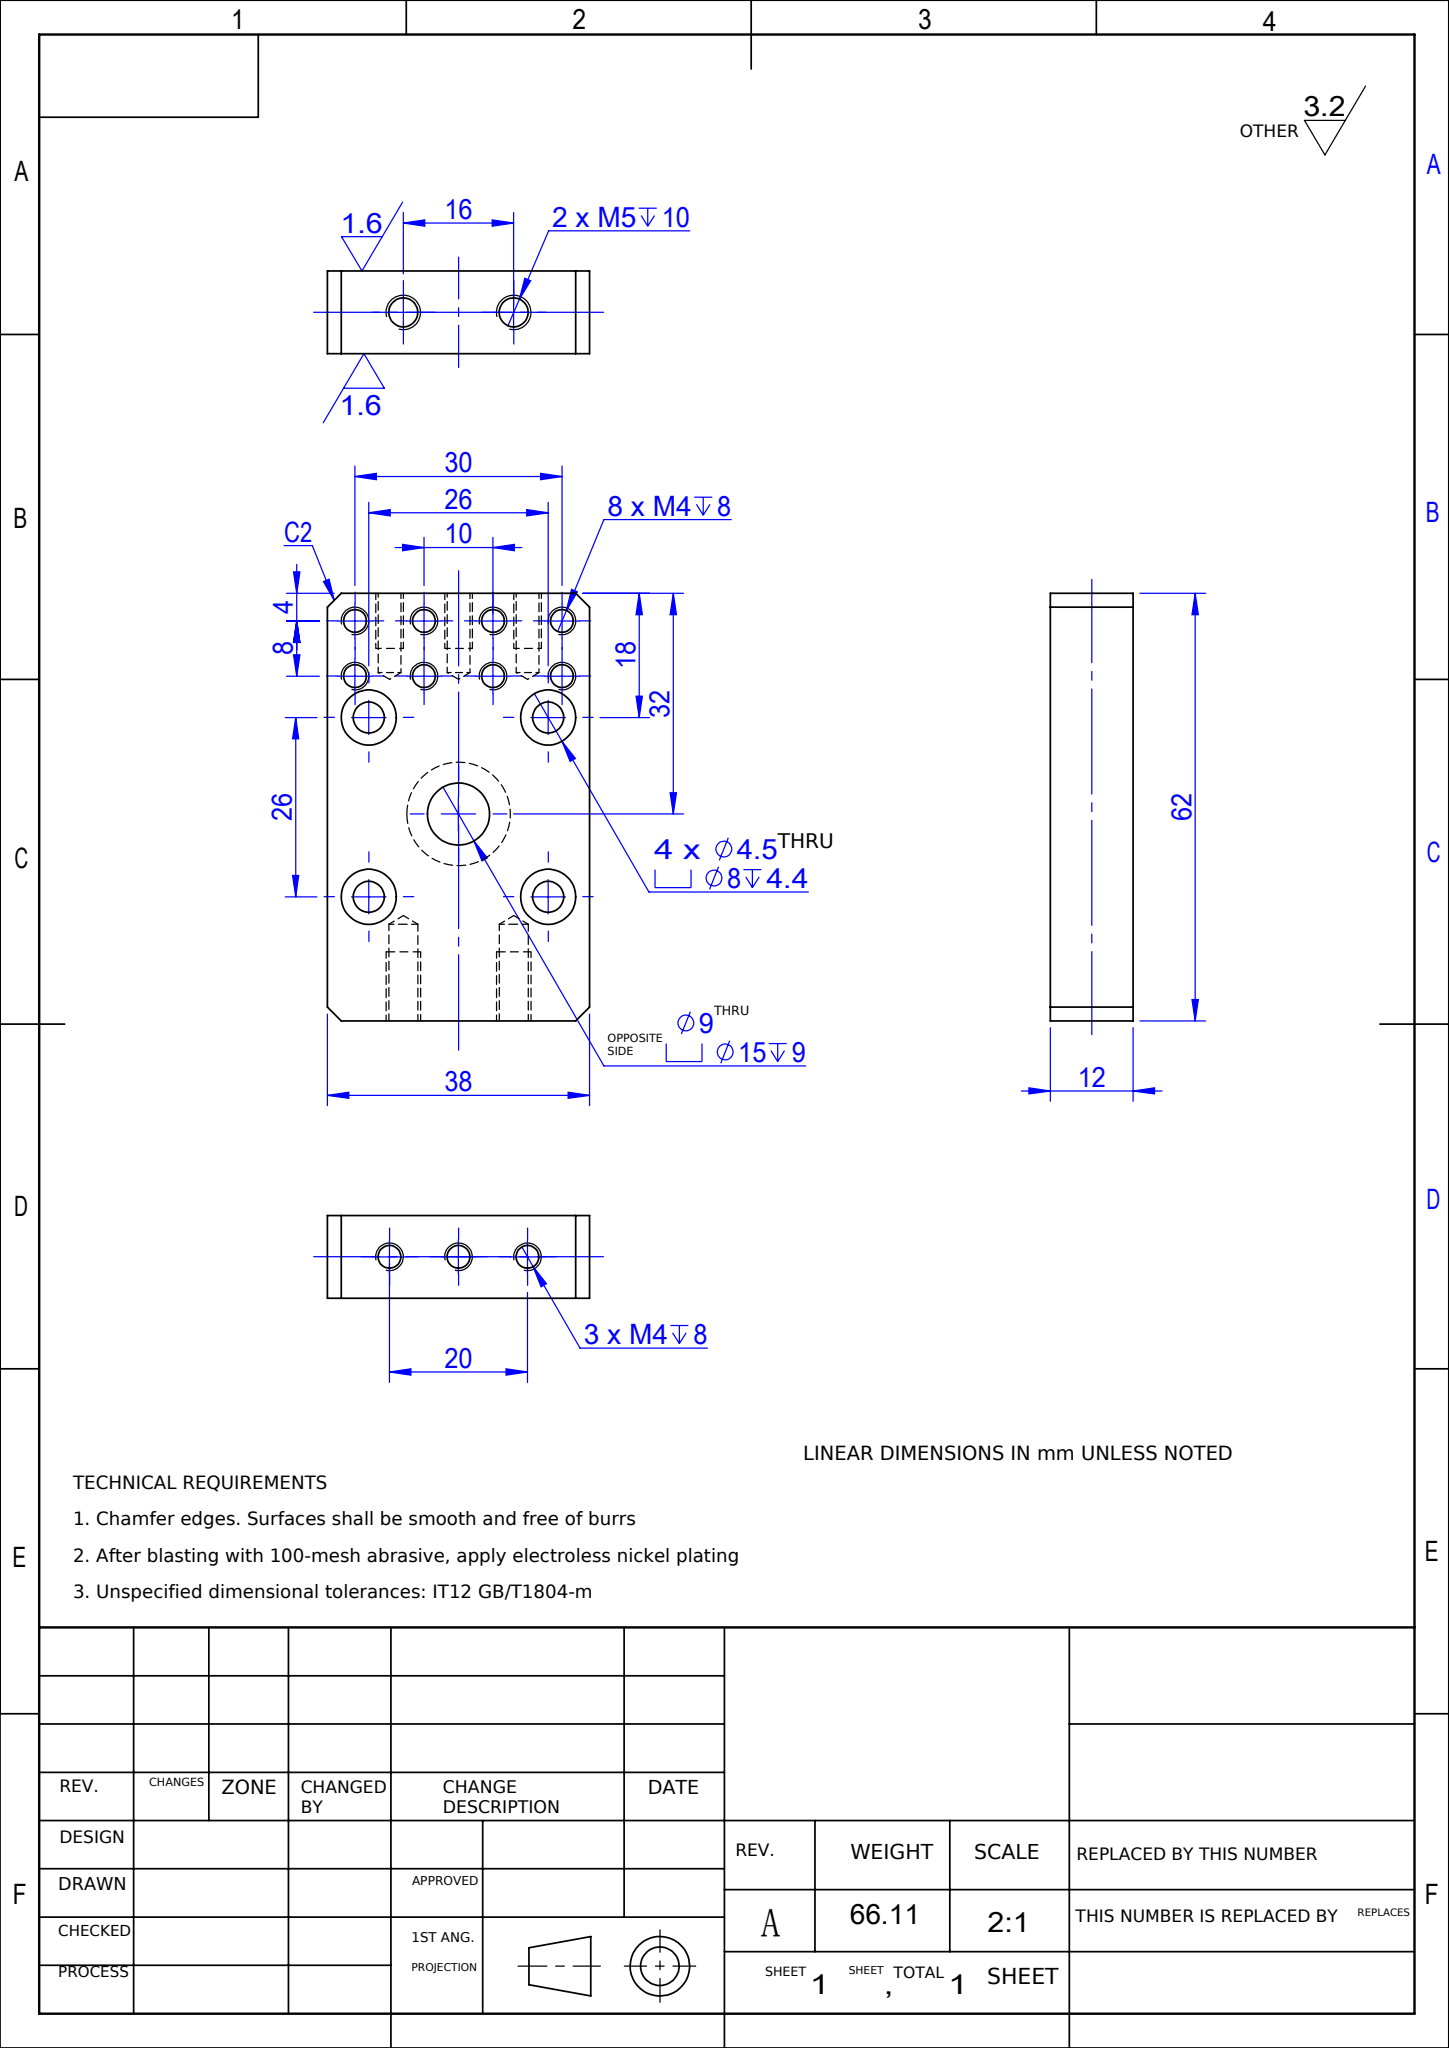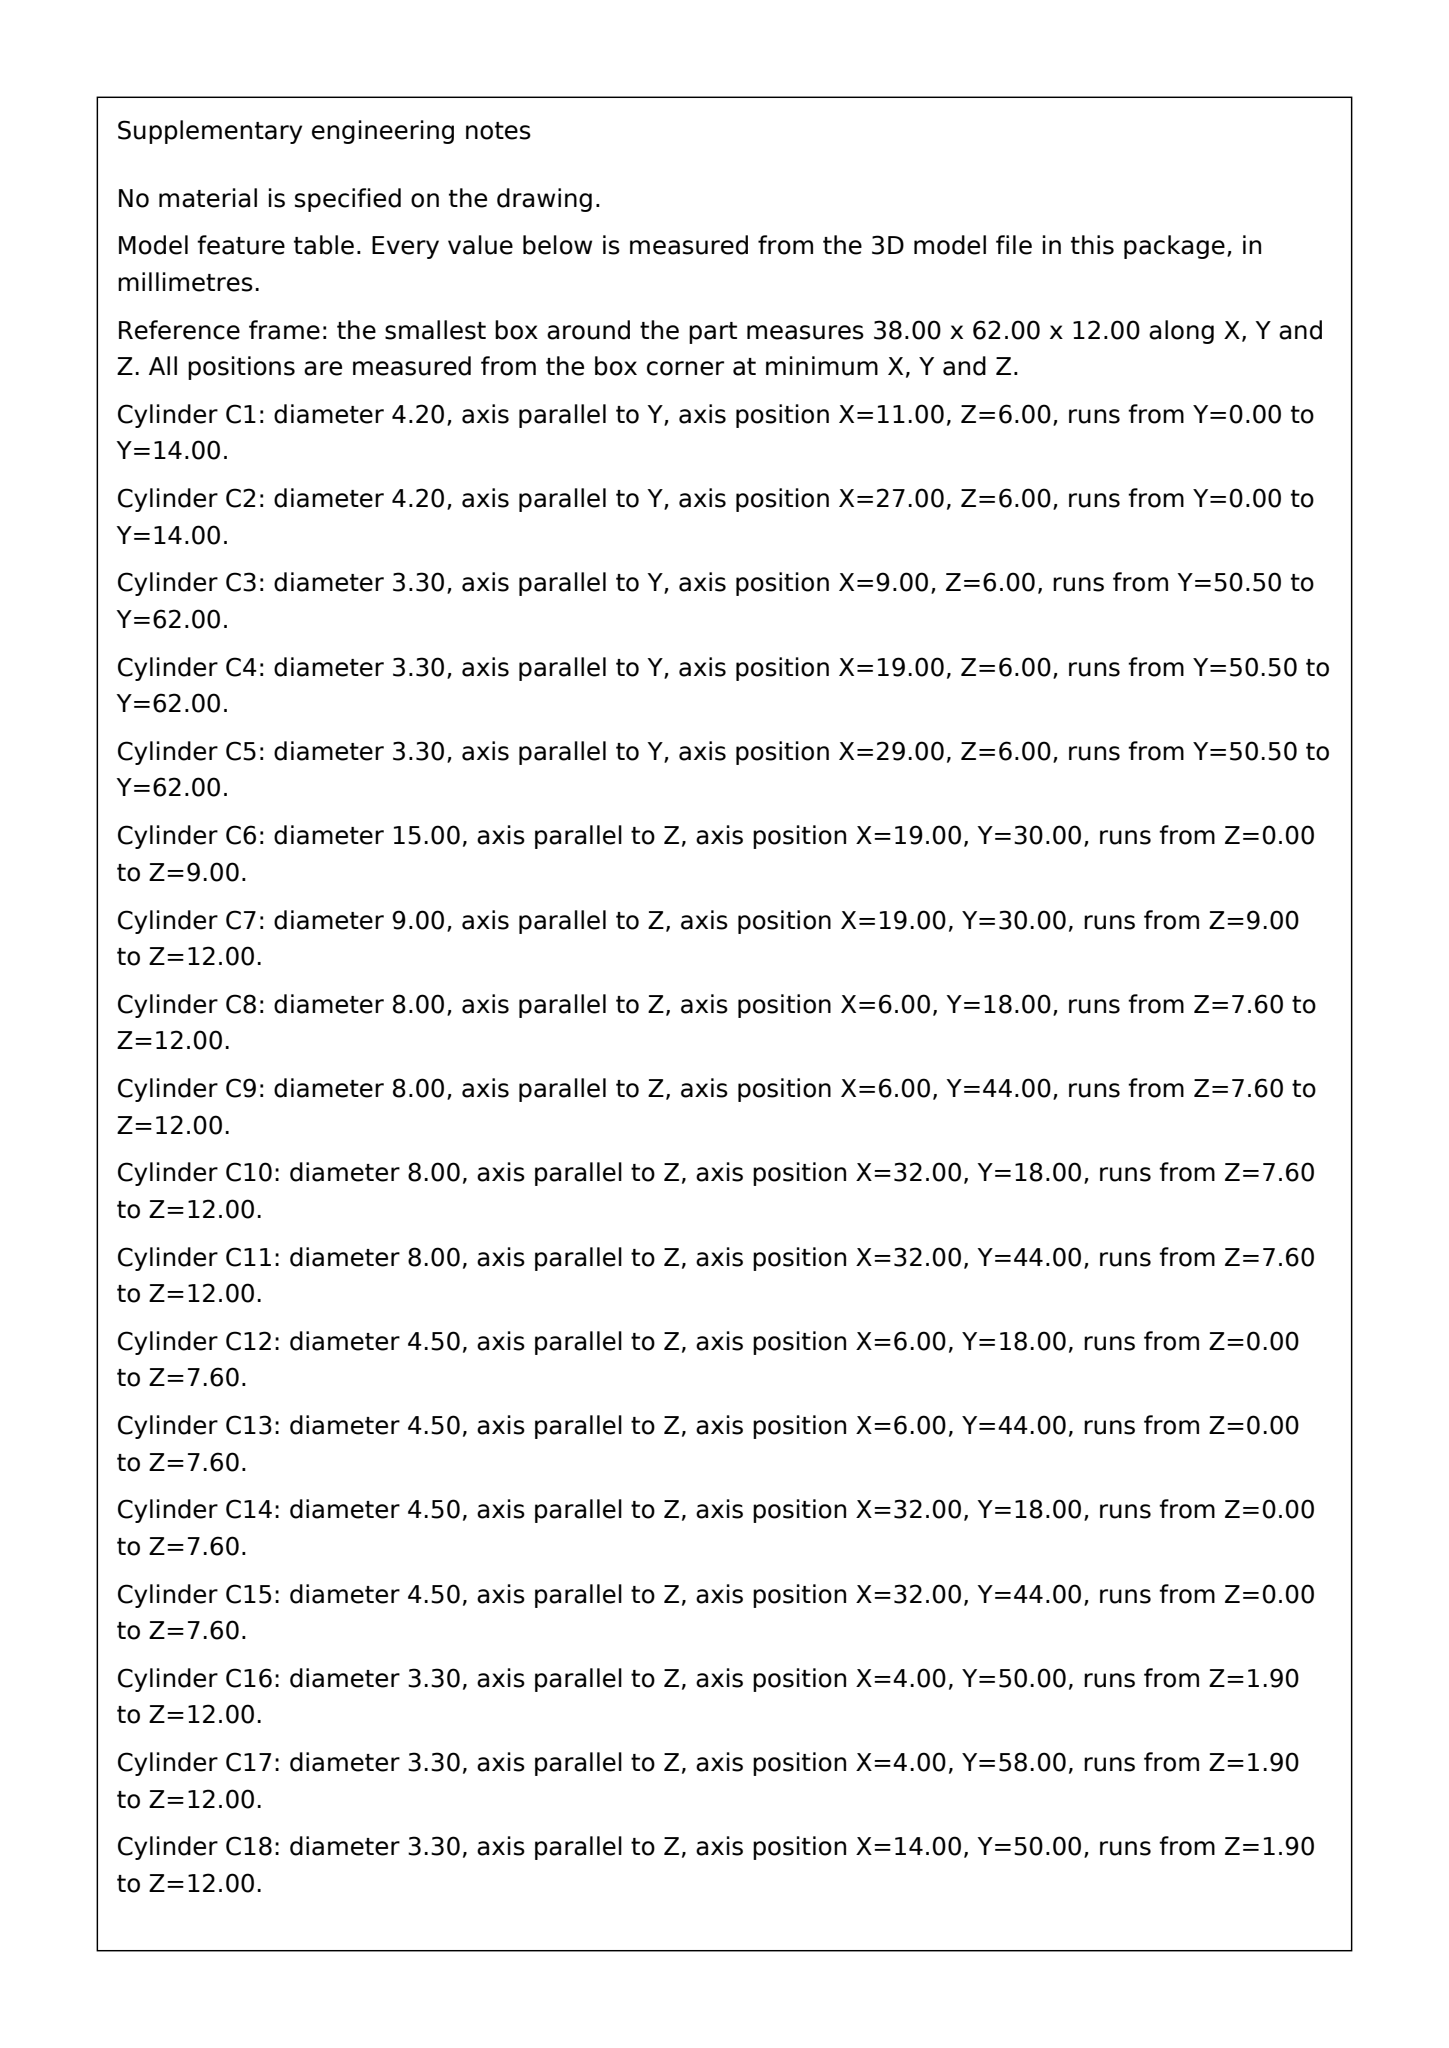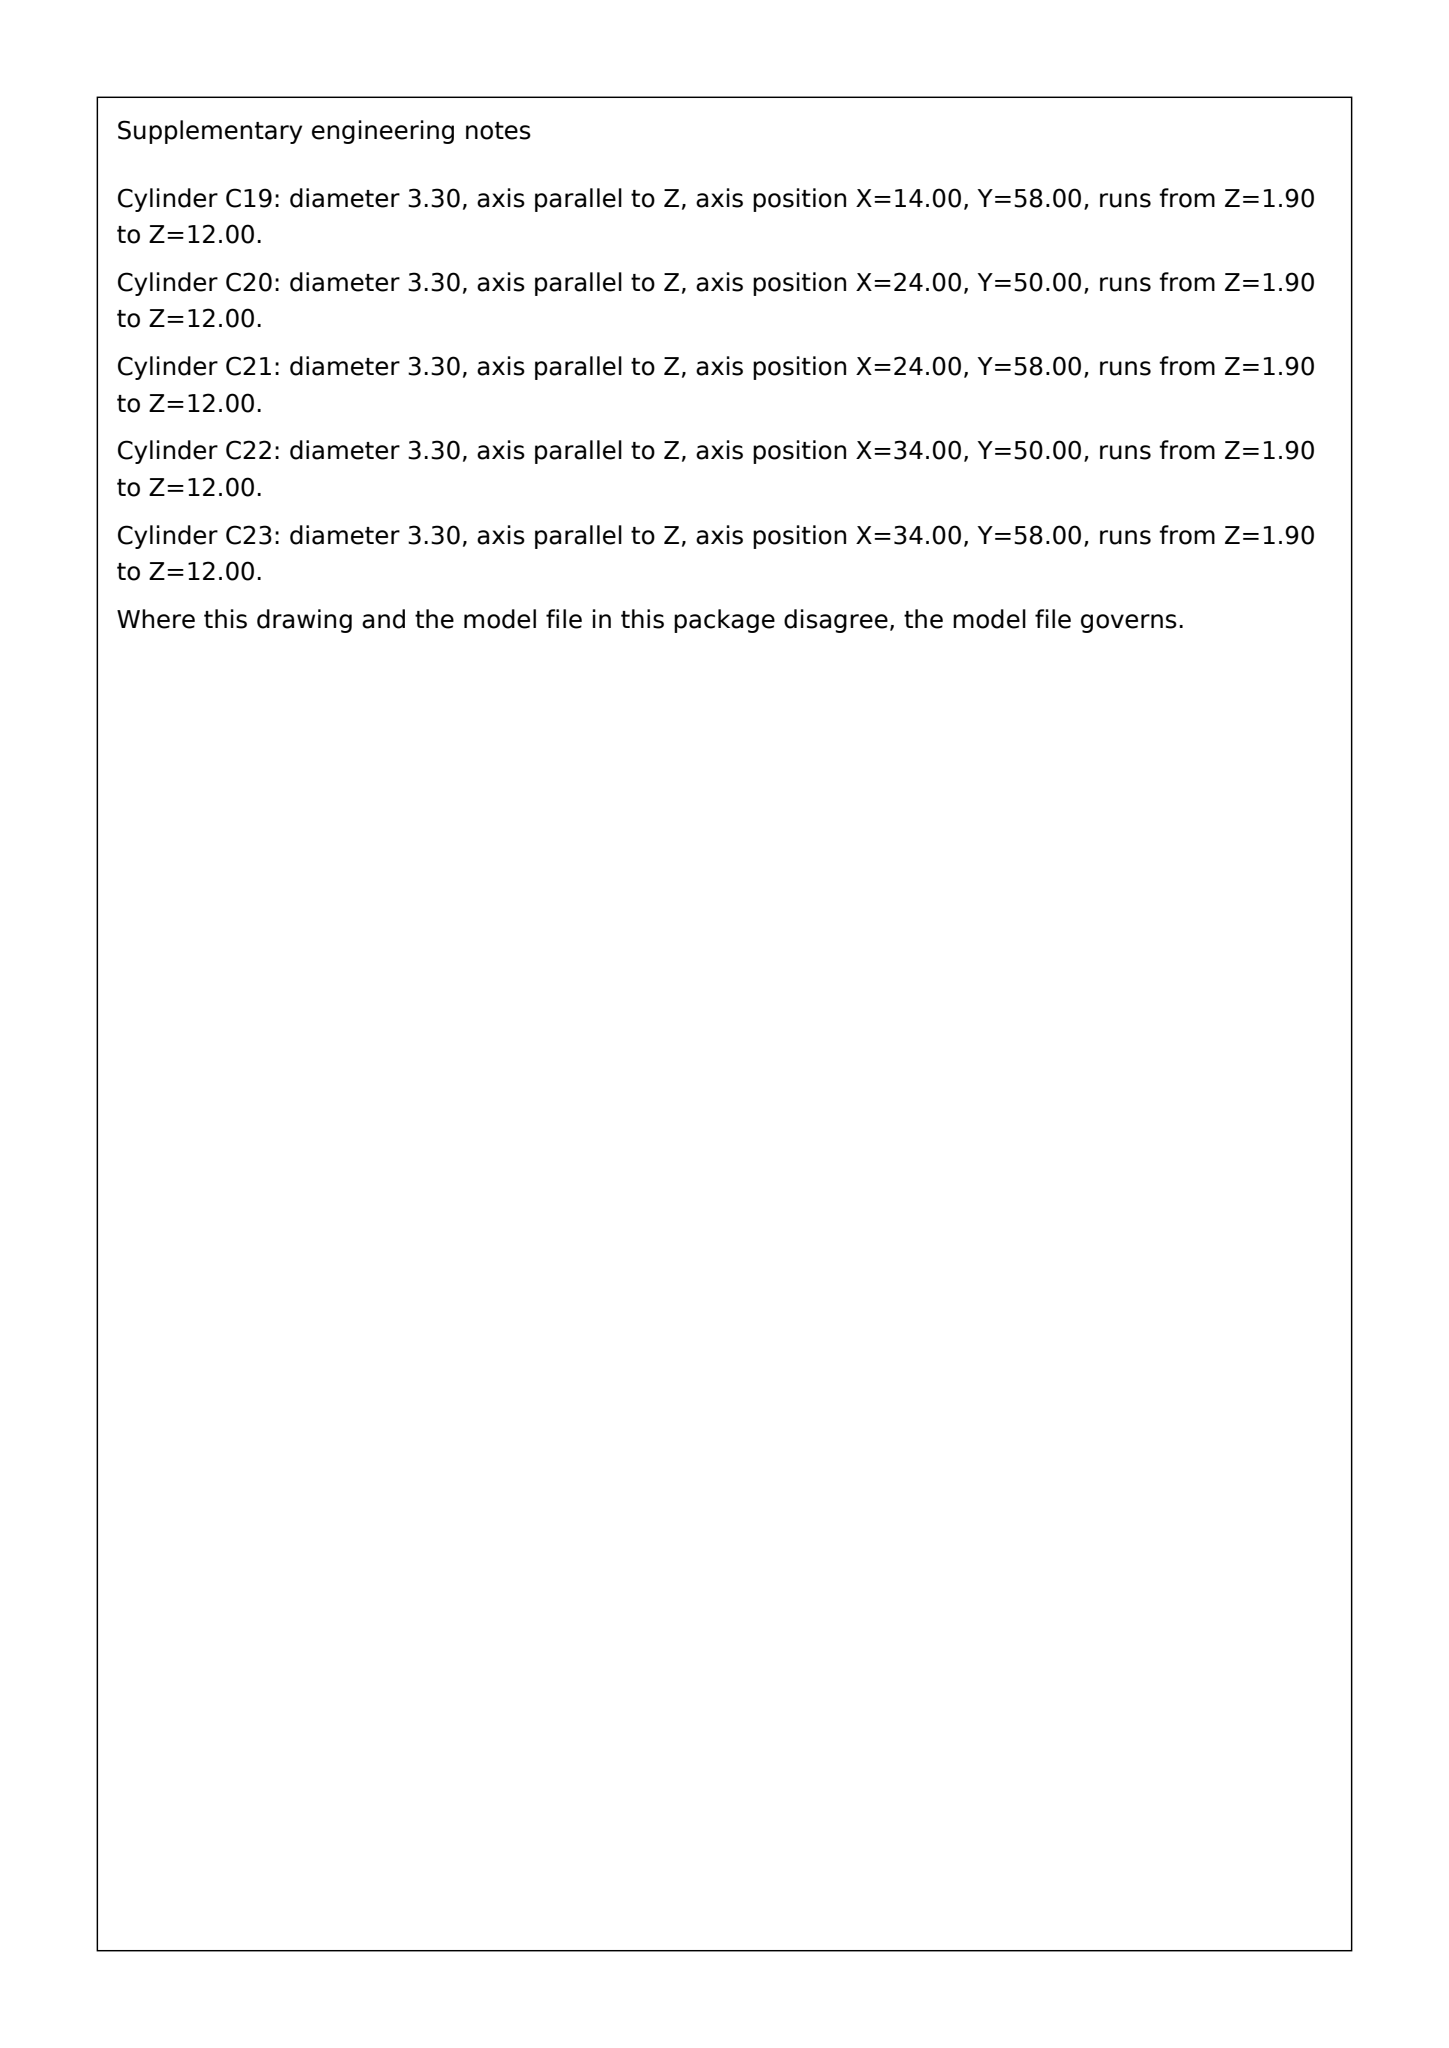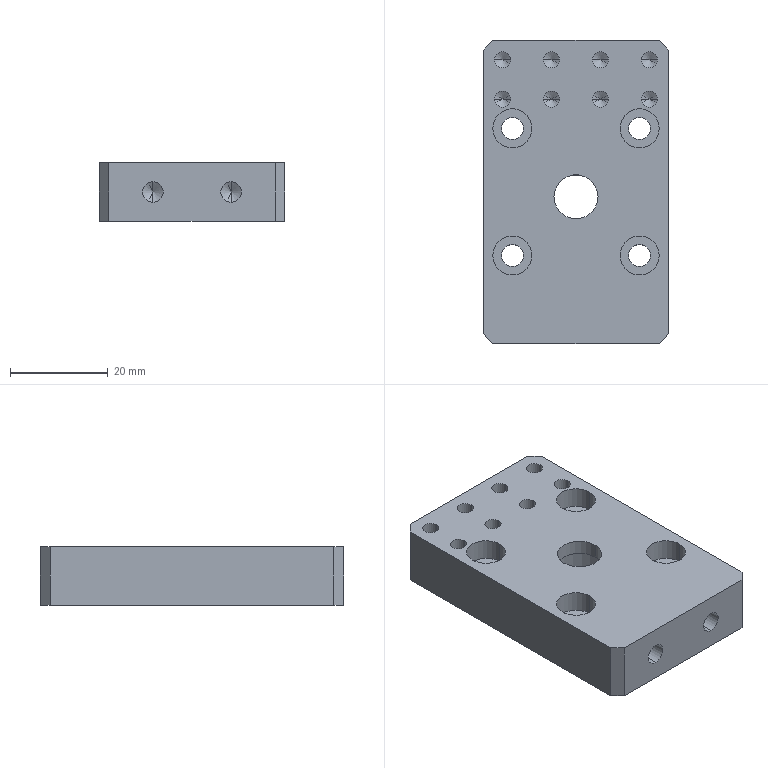Part | SolidWorks | mm | 1 solid | 87 faces | box 38 x 62 x 12 mm | volume 23610 mm3 | cylinder 46 | cone 26 | plane 15 | commonest cylinder face diameters 3.3 x22 8 x8 4.5 x8 4.2 x4 15 x2 9 x2
build123d program:
from build123d import *

# Parameters (mm, degrees)
SKETCH1_W                                       = 38
SKETCH1_H                                       = 62
BOSS_EXTRUDE1_DEPTH                             = 12
M4_HEX_SOCKET_HEAD_CAP_SCREW_CBORE2_D           = 4.5
M4_HEX_SOCKET_HEAD_CAP_SCREW_CBORE2_CBORE_D     = 8
M4_HEX_SOCKET_HEAD_CAP_SCREW_CBORE2_CBORE_DEPTH = 4.4
CHAMFER1_SIZE                                   = 2
M8_HEX_SOCKET_HEAD_CAP_SCREW_CBORE1_D           = 9
M8_HEX_SOCKET_HEAD_CAP_SCREW_CBORE1_CBORE_D     = 15
M8_HEX_SOCKET_HEAD_CAP_SCREW_CBORE1_CBORE_DEPTH = 9
M5_TAPPED_HOLE1_D                               = 4.2
M5_TAPPED_HOLE1_DEPTH                           = 14
M5_TAPPED_HOLE1_TIP                             = 1.262
M4_TAPPED_HOLE2_AT_2_COUNT                      = 2
M4_TAPPED_HOLE2_AT_2_PITCH                      = 30
M4_TAPPED_HOLE2_AT_3_COUNT                      = 2
M4_TAPPED_HOLE2_AT_3_PITCH                      = 10
M4_TAPPED_HOLE2_AT_4_COUNT                      = 2
M4_TAPPED_HOLE2_AT_4_PITCH                      = 20
M4_TAPPED_HOLE3_D                               = 3.3
M4_TAPPED_HOLE3_DEPTH                           = 11.5
M4_TAPPED_HOLE3_TIP                             = 0.9914
LPATTERN1_COUNT                                 = 2
LPATTERN1_PITCH                                 = 8


with BuildPart() as part:
    # Sketch1 → Boss-Extrude1 (new body)
    with BuildSketch(Plane.XY):
        Rectangle(SKETCH1_W, SKETCH1_H)
    extrude(amount=BOSS_EXTRUDE1_DEPTH)

    # M4 Hex Socket Head Cap Screw CBORE2 (through all)
    with Locations(Plane.XY.offset(12)):
        with Locations((-13, 13), (13, 13), (-13, -13), (13, -13)):
            CounterBoreHole(M4_HEX_SOCKET_HEAD_CAP_SCREW_CBORE2_D / 2, M4_HEX_SOCKET_HEAD_CAP_SCREW_CBORE2_CBORE_D / 2, M4_HEX_SOCKET_HEAD_CAP_SCREW_CBORE2_CBORE_DEPTH)

    # Chamfer1
    chamfer1_edges = [part.edges().sort_by_distance(p)[0] for p in [
        (19, -31, 6),
        (-19, -31, 6),
        (-19, 31, 6),
        (19, 31, 6),
    ]]
    chamfer(chamfer1_edges, length=CHAMFER1_SIZE)

    # M8 Hex Socket Head Cap Screw CBORE1 (through all)
    with Locations(Plane(origin=(0, 0, 0), x_dir=(-1, 0, 0), z_dir=(0, 0, -1))):
        with Locations((0, -1)):
            CounterBoreHole(M8_HEX_SOCKET_HEAD_CAP_SCREW_CBORE1_D / 2, M8_HEX_SOCKET_HEAD_CAP_SCREW_CBORE1_CBORE_D / 2, M8_HEX_SOCKET_HEAD_CAP_SCREW_CBORE1_CBORE_DEPTH)

    # M5 Tapped Hole1
    with Locations(Plane.XZ.offset(31)):
        with Locations((8, 6), (-8, 6)):
            Hole(M5_TAPPED_HOLE1_D / 2, depth=M5_TAPPED_HOLE1_DEPTH)
            with Locations((0, 0, -(M5_TAPPED_HOLE1_DEPTH + M5_TAPPED_HOLE1_TIP / 2))):  # 118° drill point
                Cone(0, M5_TAPPED_HOLE1_D / 2, M5_TAPPED_HOLE1_TIP, mode=Mode.SUBTRACT)

    # Sketch19 → M4 Tapped Hole2 (revolve, cut)
    with BuildSketch(Plane(origin=(-15, 19, 12), x_dir=(0, -1, 0), z_dir=(1, 0, 0))):
        Polygon((0, 0), (0, 11.091), (1.65, 10.1), (1.65, 0), align=None)
    m4_tapped_hole2 = revolve(axis=Axis((-15, 19, 18.35), (0, 0, -1)), mode=Mode.SUBTRACT)

    # M4 Tapped Hole2 at 2: M4 Tapped Hole2 ×2
    with Locations(*[(i * M4_TAPPED_HOLE2_AT_2_PITCH, 0, 0) for i in range(1, M4_TAPPED_HOLE2_AT_2_COUNT)]):
        add(m4_tapped_hole2, mode=Mode.SUBTRACT)

    # M4 Tapped Hole2 at 3: M4 Tapped Hole2 ×2
    with Locations(*[(i * M4_TAPPED_HOLE2_AT_3_PITCH, 0, 0) for i in range(1, M4_TAPPED_HOLE2_AT_3_COUNT)]):
        add(m4_tapped_hole2, mode=Mode.SUBTRACT)

    # M4 Tapped Hole2 at 4: M4 Tapped Hole2 ×2
    with Locations(*[(i * M4_TAPPED_HOLE2_AT_4_PITCH, 0, 0) for i in range(1, M4_TAPPED_HOLE2_AT_4_COUNT)]):
        add(m4_tapped_hole2, mode=Mode.SUBTRACT)

    # M4 Tapped Hole3
    with Locations(Plane(origin=(0, 31, 0), x_dir=(-1, 0, 0), z_dir=(0, 1, 0))):
        with Locations((10, 6), (-10, 6), (0, 6)):
            Hole(M4_TAPPED_HOLE3_D / 2, depth=M4_TAPPED_HOLE3_DEPTH)
            with Locations((0, 0, -(M4_TAPPED_HOLE3_DEPTH + M4_TAPPED_HOLE3_TIP / 2))):  # 118° drill point
                Cone(0, M4_TAPPED_HOLE3_D / 2, M4_TAPPED_HOLE3_TIP, mode=Mode.SUBTRACT)

    # LPattern1: M4 Tapped Hole2 ×2
    with Locations(*[(0, i * LPATTERN1_PITCH, 0) for i in range(1, LPATTERN1_COUNT)]):
        add(m4_tapped_hole2, mode=Mode.SUBTRACT)

    # LPattern1 copy 1 sketch → LPattern1 copy 1 (revolve, cut)
    with BuildSketch(Plane(origin=(15, 27, 12), x_dir=(0, -1, 0), z_dir=(1, 0, 0))):
        Polygon((0, 0), (0, 11.091), (1.65, 10.1), (1.65, 0), align=None)
    revolve(axis=Axis((15, 27, 18.35), (0, 0, -1)), mode=Mode.SUBTRACT)

    # LPattern1 copy 2 sketch → LPattern1 copy 2 (revolve, cut)
    with BuildSketch(Plane(origin=(-5, 27, 12), x_dir=(0, -1, 0), z_dir=(1, 0, 0))):
        Polygon((0, 0), (0, 11.091), (1.65, 10.1), (1.65, 0), align=None)
    revolve(axis=Axis((-5, 27, 18.35), (0, 0, -1)), mode=Mode.SUBTRACT)

    # LPattern1 copy 3 sketch → LPattern1 copy 3 (revolve, cut)
    with BuildSketch(Plane(origin=(5, 27, 12), x_dir=(0, -1, 0), z_dir=(1, 0, 0))):
        Polygon((0, 0), (0, 11.091), (1.65, 10.1), (1.65, 0), align=None)
    revolve(axis=Axis((5, 27, 18.35), (0, 0, -1)), mode=Mode.SUBTRACT)


solid = part.part